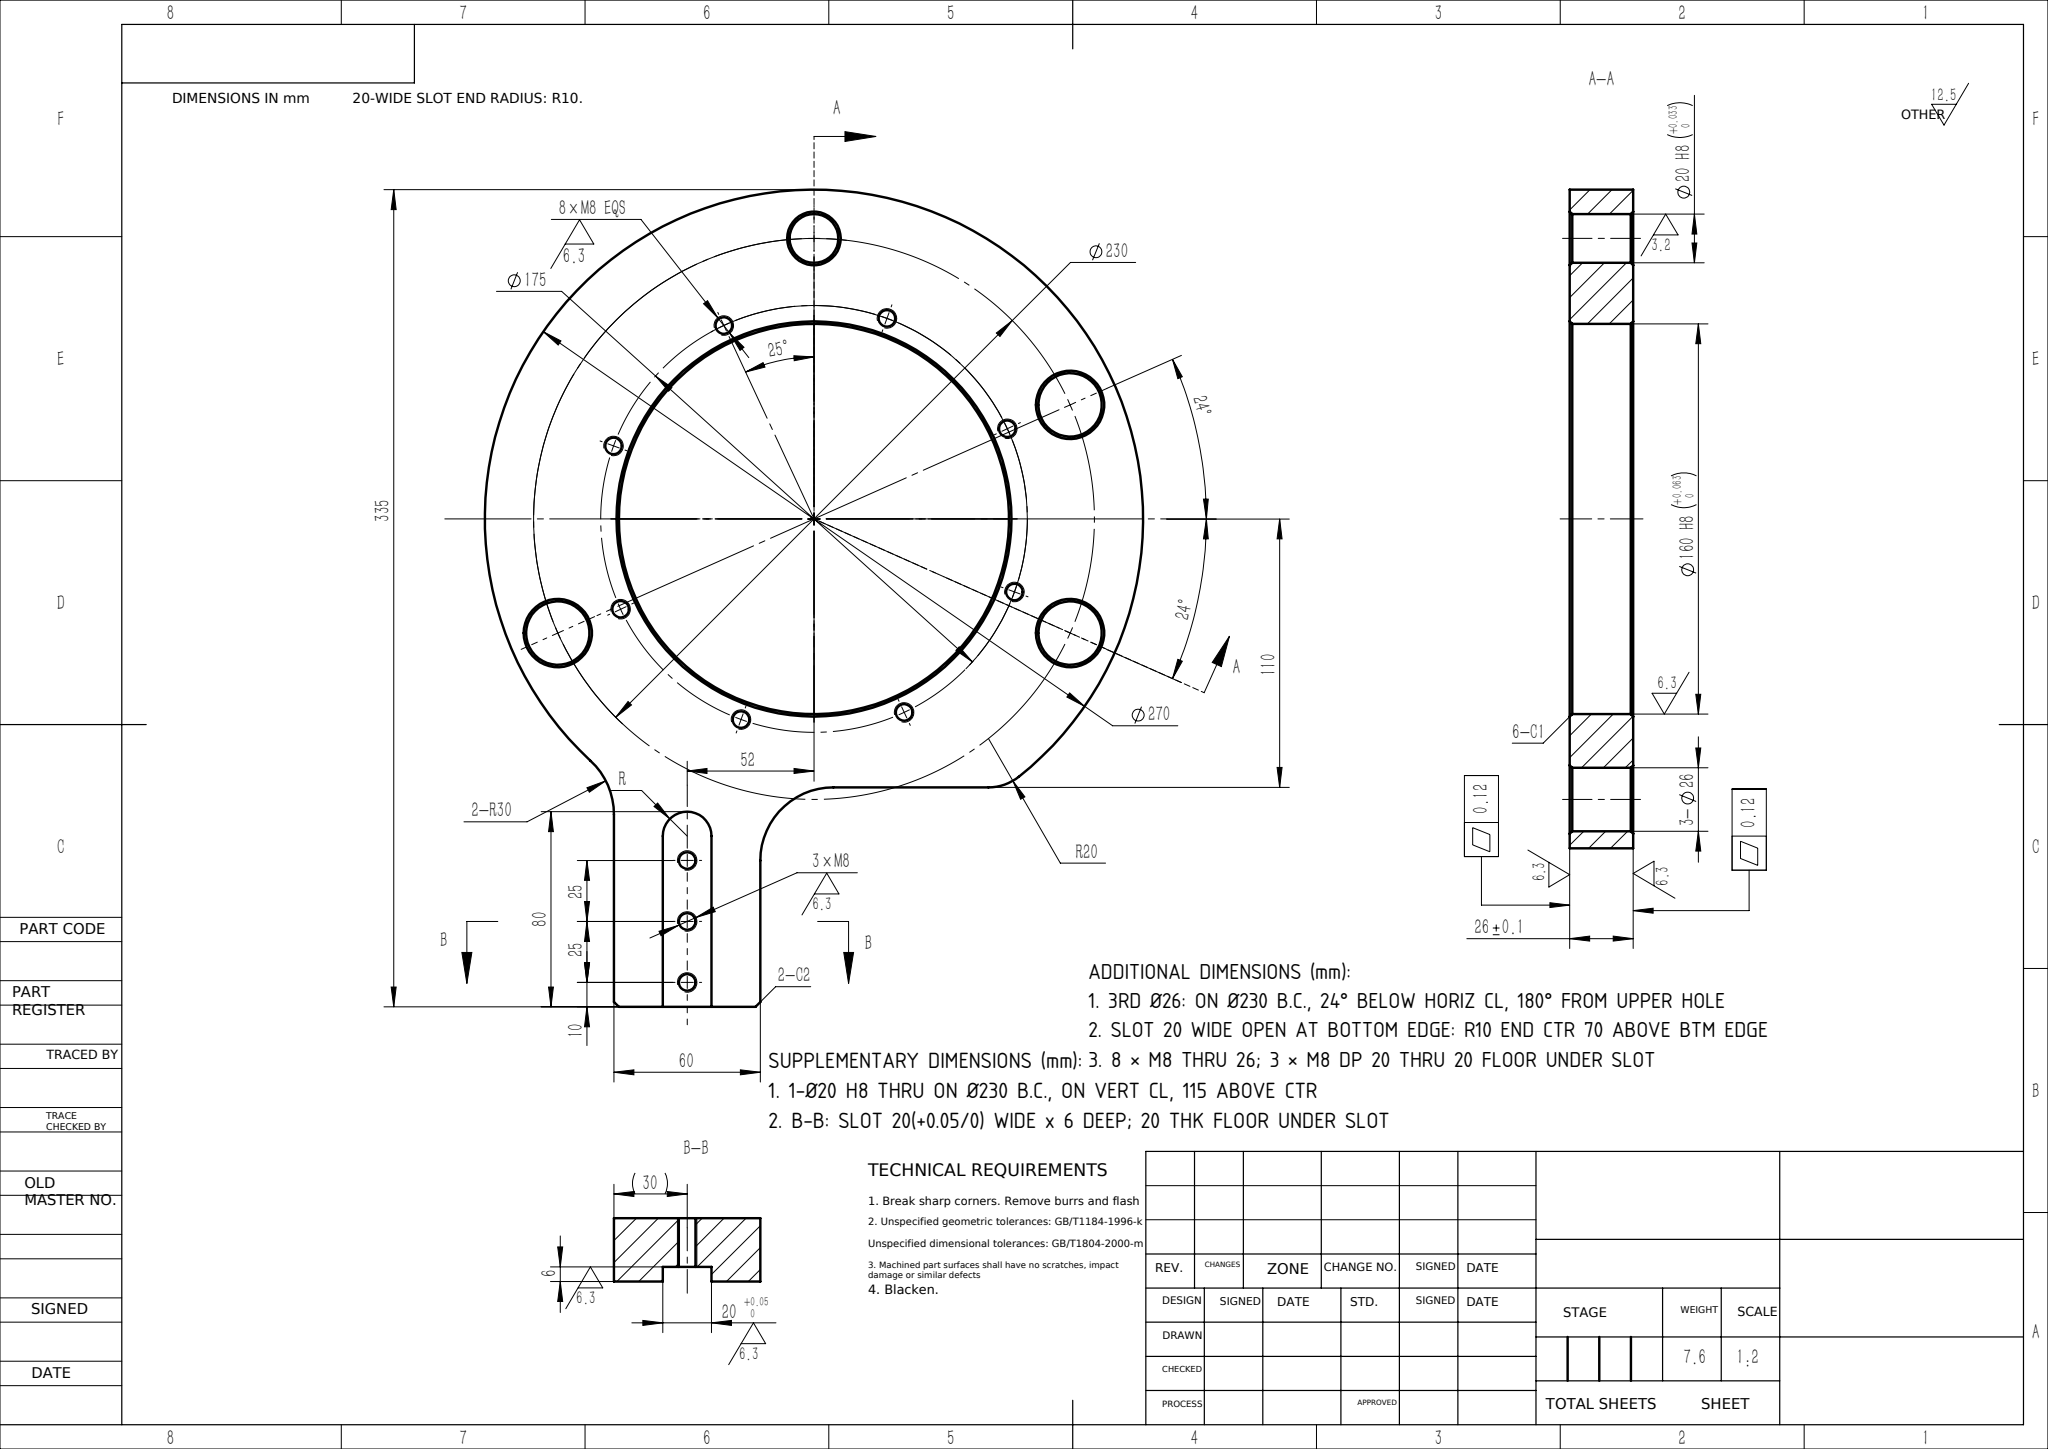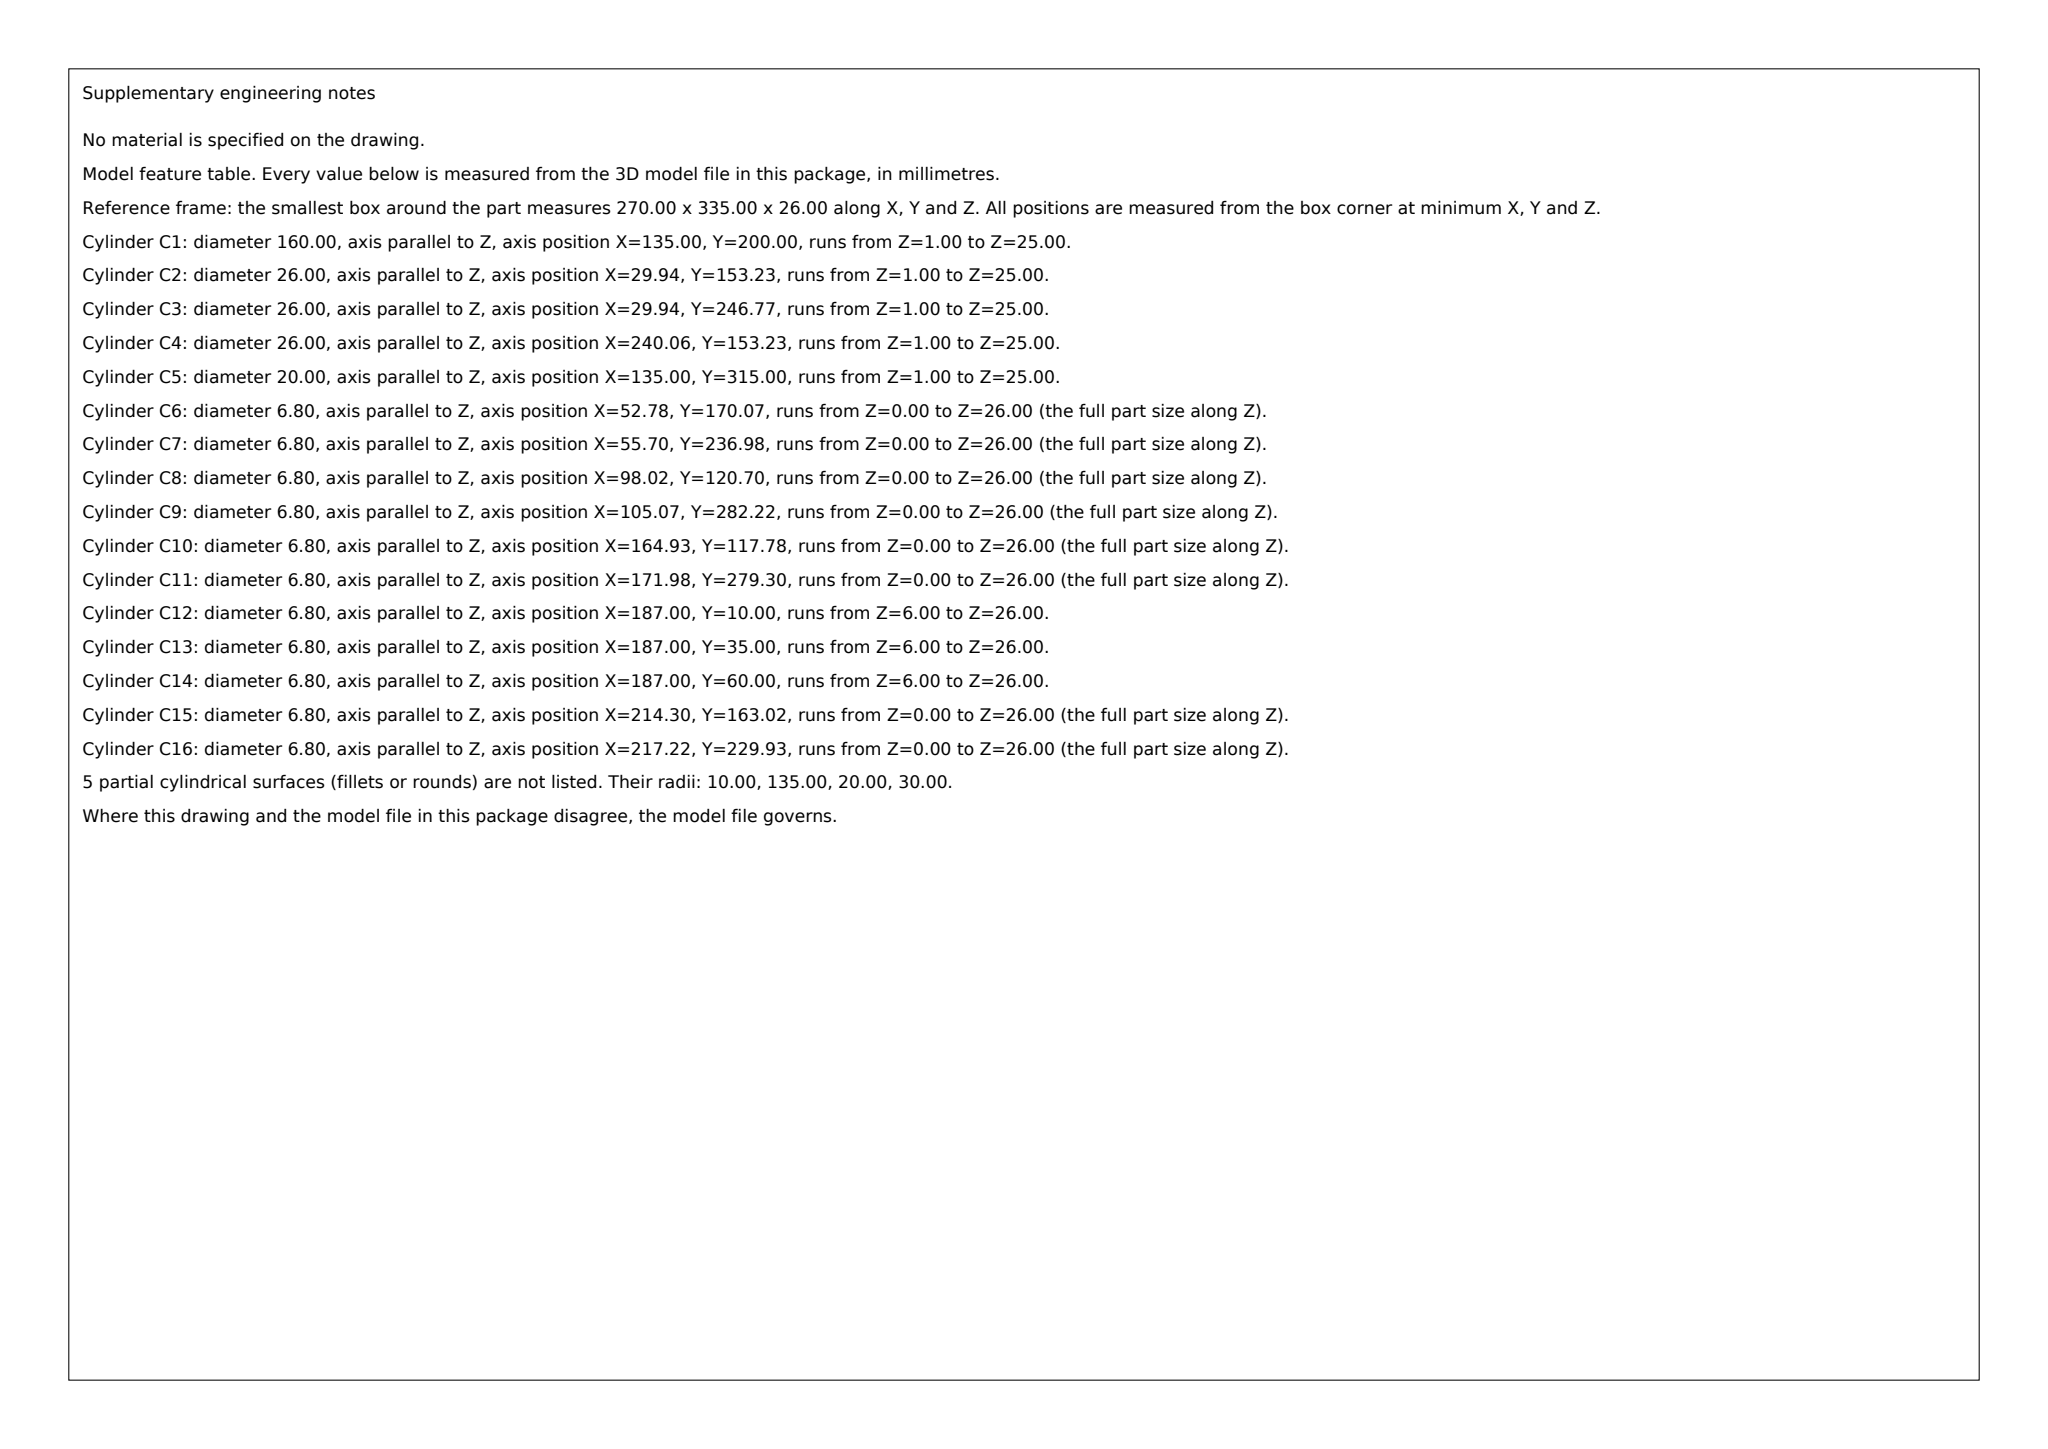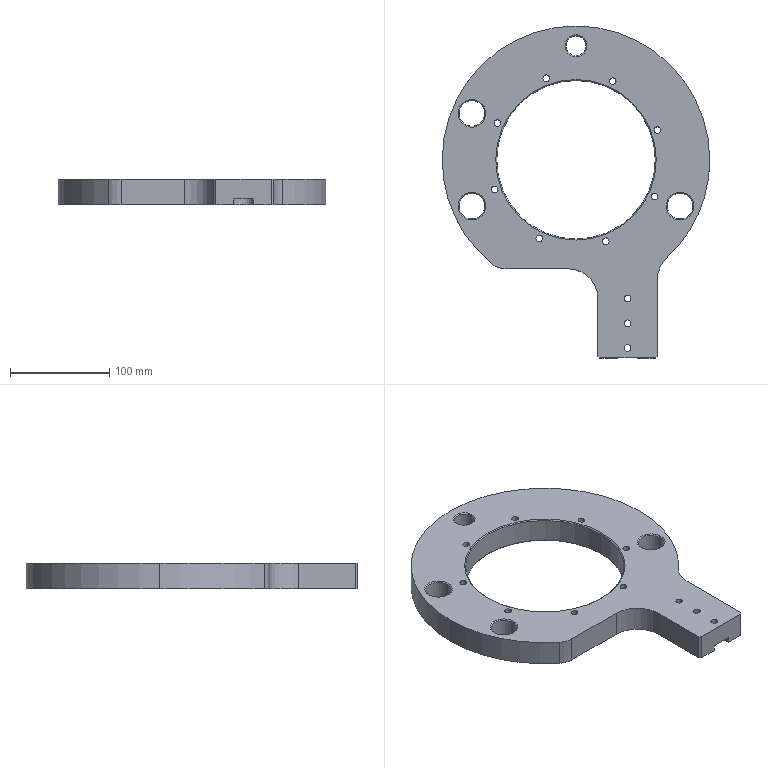Part | SolidWorks | mm | 1 solid | 70 faces | box 270 x 335 x 26 mm | volume 973192 mm3 | cylinder 39 | cone 20 | plane 11 | commonest cylinder face diameters 6.8 x22 26 x6 20 x3 270 x3 160 x2 60 x2 40 x1